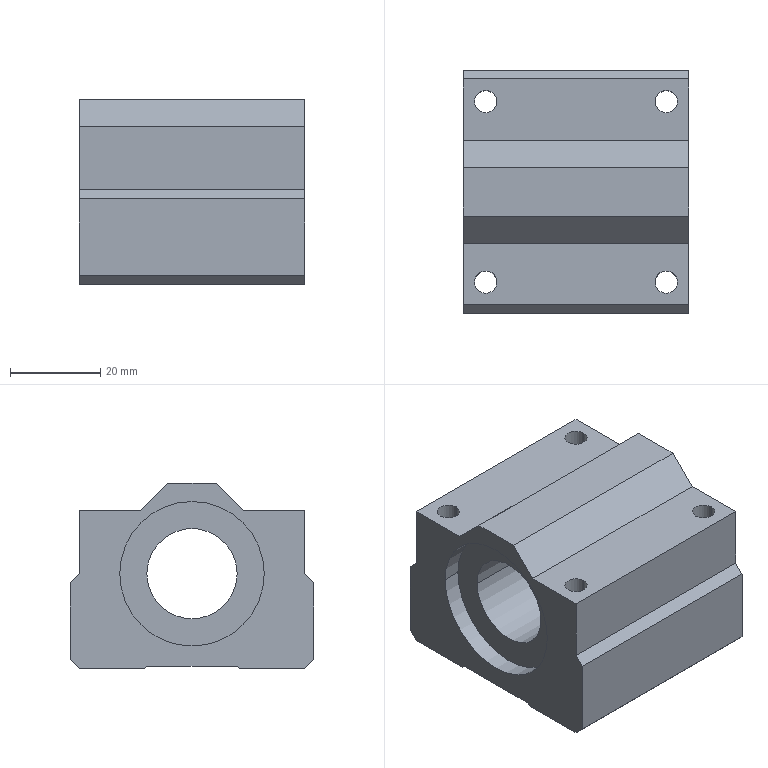Component | SolidWorks | LMW01-d20-1 | 1 solid | 44 faces | volume 73531 mm3 | plane 22 | cylinder 14 | cone 8 | commonest cylinder face diameters 4.917 x8 32 x4 20 x2